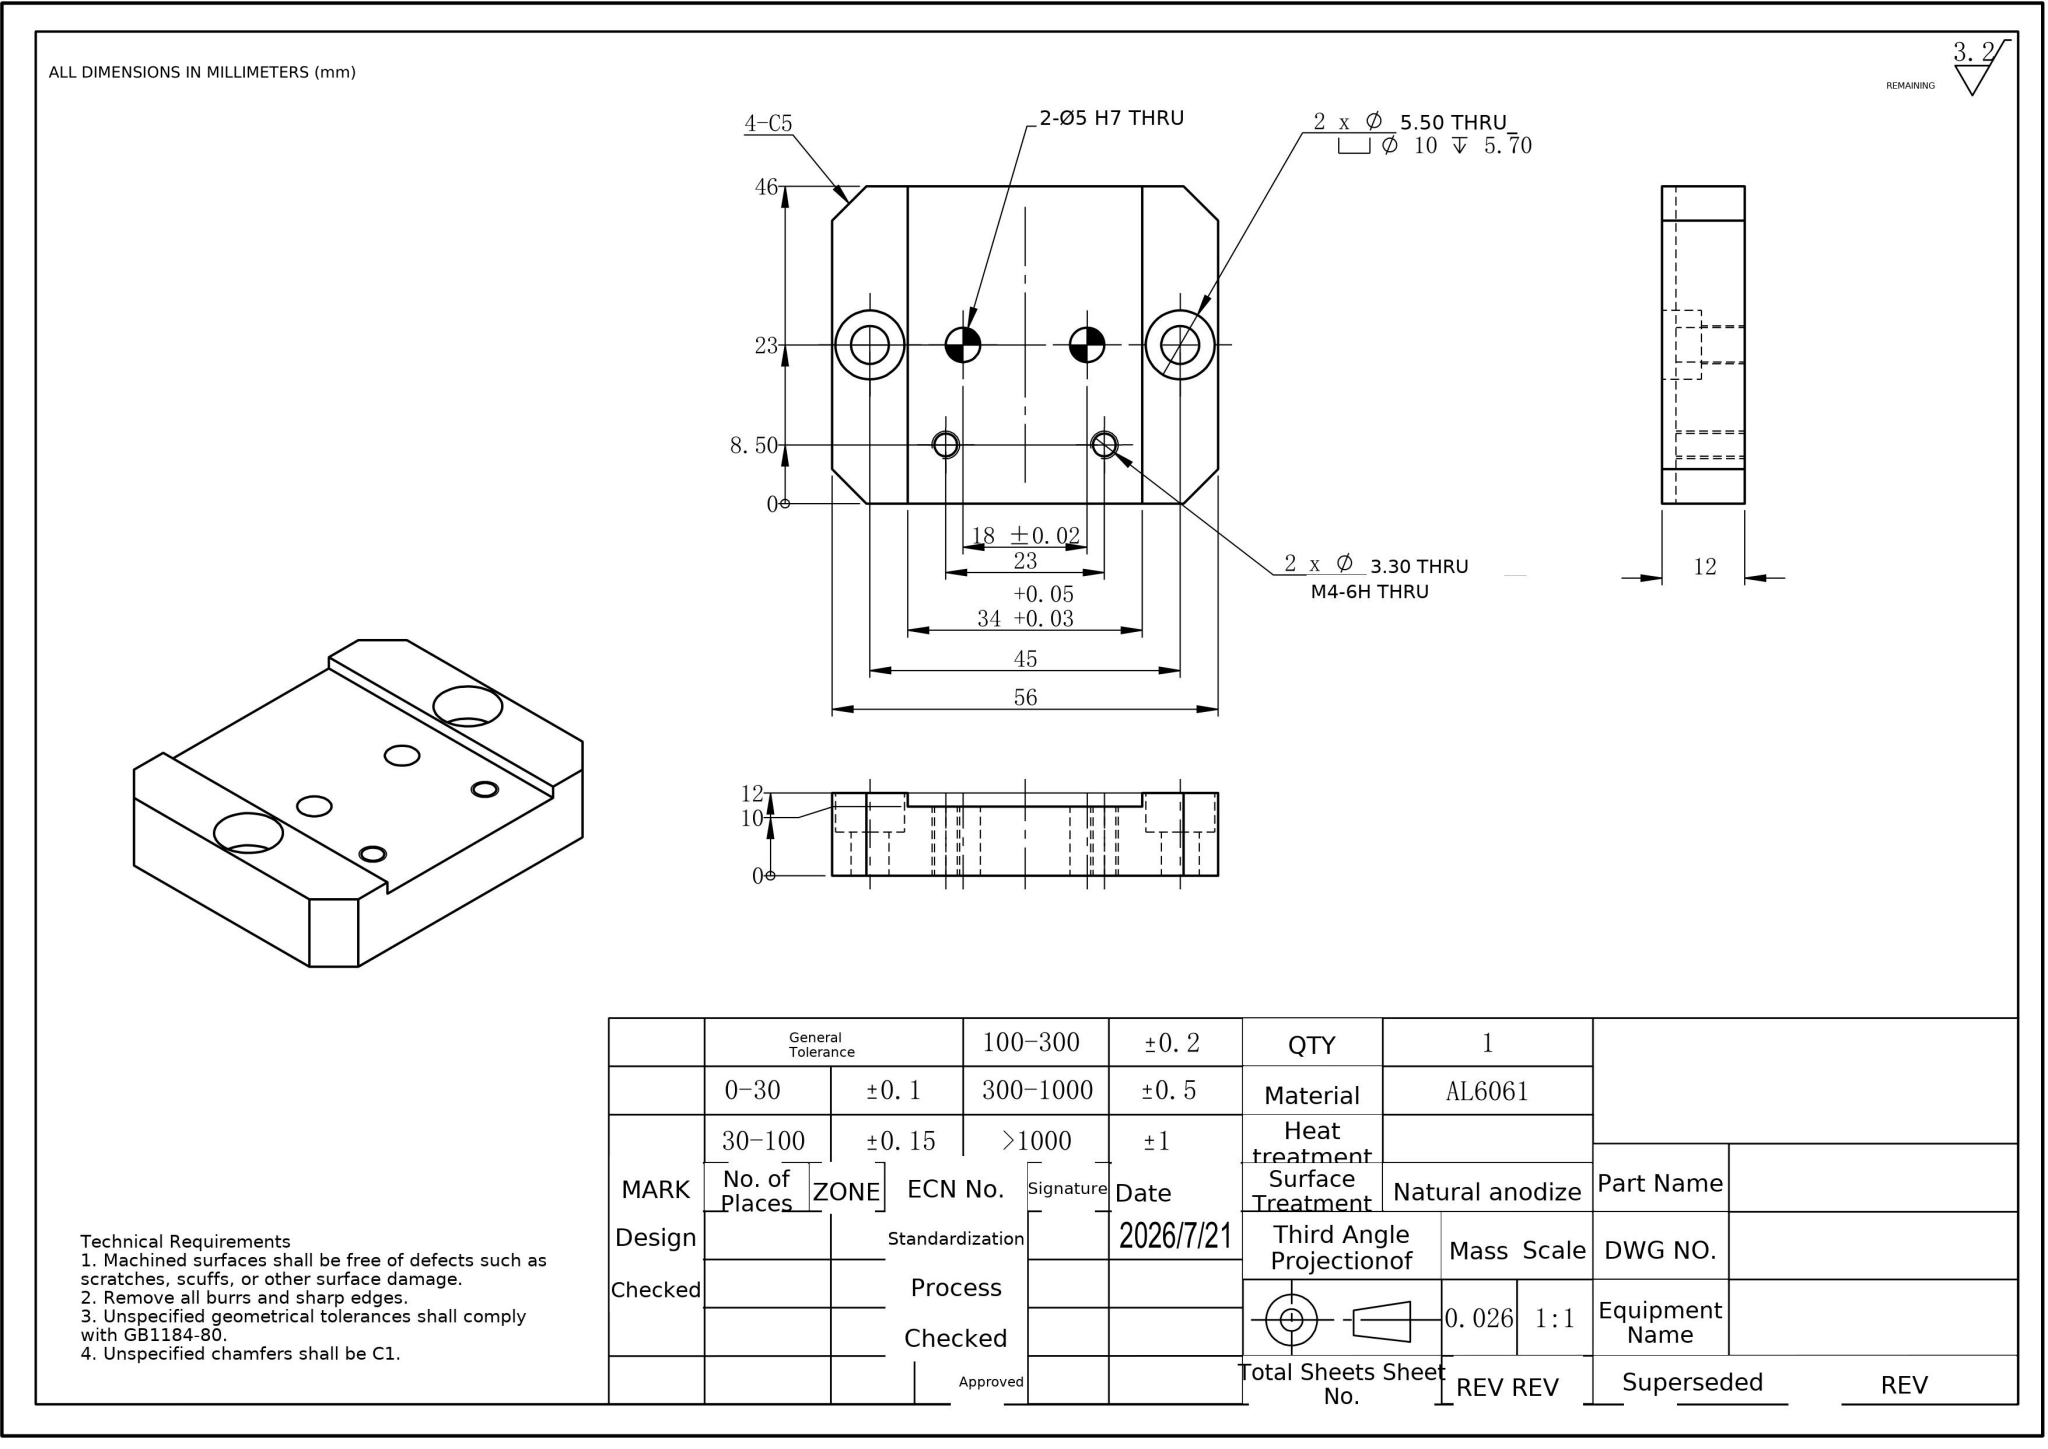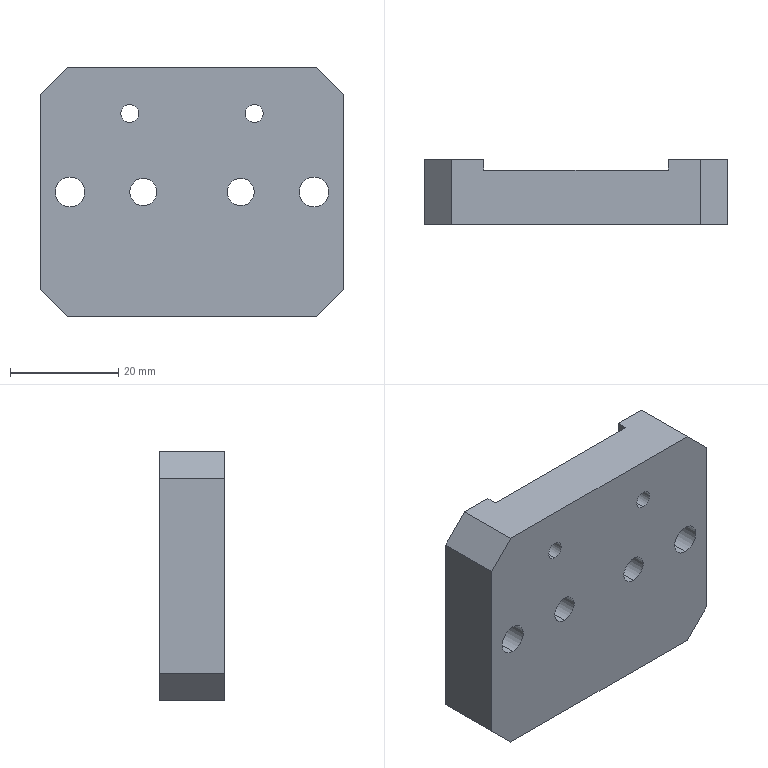Part | NX | mm | 1 solid | 32 faces | box 56 x 12 x 46 mm | volume 25426 mm3 | cylinder 16 | plane 16 | commonest cylinder face diameters 3.3 x4 5 x4 10 x4 5.5 x4
STEP:
#1=COLOUR_RGB('',0.7922,0.8196,0.9333);
#2=FILL_AREA_STYLE_COLOUR('',#1);
#3=FILL_AREA_STYLE('',(#2));
#4=SURFACE_STYLE_FILL_AREA(#3);
#5=SURFACE_SIDE_STYLE('',(#4));
#6=SURFACE_STYLE_USAGE(.BOTH.,#5);
#7=PRESENTATION_STYLE_ASSIGNMENT((#6));
#8=CARTESIAN_POINT('',(11.5,-5.,12.85));
#9=VERTEX_POINT('',#8);
#10=CARTESIAN_POINT('',(11.5,-5.,16.15));
#11=VERTEX_POINT('',#10);
#12=CARTESIAN_POINT('',(11.5,-5.,14.5));
#13=DIRECTION('',(0.,1.,0.));
#14=DIRECTION('',(0.,0.,1.));
#15=AXIS2_PLACEMENT_3D('',#12,#13,#14);
#16=CIRCLE('',#15,1.65);
#17=EDGE_CURVE('',#9,#11,#16,.T.);
#18=ORIENTED_EDGE('',*,*,#17,.F.);
#19=CARTESIAN_POINT('',(11.5,5.,12.85));
#20=VERTEX_POINT('',#19);
#21=CARTESIAN_POINT('',(11.5,7.,12.85));
#22=DIRECTION('',(0.,1.,0.));
#23=VECTOR('',#22,1000.);
#24=LINE('',#21,#23);
#25=EDGE_CURVE('',#9,#20,#24,.T.);
#26=ORIENTED_EDGE('',*,*,#25,.T.);
#27=CARTESIAN_POINT('',(11.5,5.,16.15));
#28=VERTEX_POINT('',#27);
#29=CARTESIAN_POINT('',(11.5,5.,14.5));
#30=DIRECTION('',(0.,-1.,0.));
#31=DIRECTION('',(0.,0.,-1.));
#32=AXIS2_PLACEMENT_3D('',#29,#30,#31);
#33=CIRCLE('',#32,1.65);
#34=EDGE_CURVE('',#28,#20,#33,.T.);
#35=ORIENTED_EDGE('',*,*,#34,.F.);
#36=CARTESIAN_POINT('',(11.5,7.,16.15));
#37=DIRECTION('',(0.,1.,0.));
#38=VECTOR('',#37,1000.);
#39=LINE('',#36,#38);
#40=EDGE_CURVE('',#11,#28,#39,.T.);
#41=ORIENTED_EDGE('',*,*,#40,.F.);
#42=EDGE_LOOP('',(#18,#26,#35,#41));
#43=FACE_OUTER_BOUND('',#42,.T.);
#44=CARTESIAN_POINT('',(11.5,7.,14.5));
#45=DIRECTION('',(0.,1.,0.));
#46=DIRECTION('',(0.,0.,1.));
#47=AXIS2_PLACEMENT_3D('',#44,#45,#46);
#48=CYLINDRICAL_SURFACE('',#47,1.65);
#49=ADVANCED_FACE('',(#43),#48,.F.);
#50=CARTESIAN_POINT('',(-11.5,-5.,12.85));
#51=VERTEX_POINT('',#50);
#52=CARTESIAN_POINT('',(-11.5,-5.,16.15));
#53=VERTEX_POINT('',#52);
#54=CARTESIAN_POINT('',(-11.5,-5.,14.5));
#55=DIRECTION('',(0.,1.,0.));
#56=DIRECTION('',(0.,0.,1.));
#57=AXIS2_PLACEMENT_3D('',#54,#55,#56);
#58=CIRCLE('',#57,1.65);
#59=EDGE_CURVE('',#51,#53,#58,.T.);
#60=ORIENTED_EDGE('',*,*,#59,.F.);
#61=CARTESIAN_POINT('',(-11.5,5.,12.85));
#62=VERTEX_POINT('',#61);
#63=CARTESIAN_POINT('',(-11.5,7.,12.85));
#64=DIRECTION('',(0.,1.,0.));
#65=VECTOR('',#64,1000.);
#66=LINE('',#63,#65);
#67=EDGE_CURVE('',#51,#62,#66,.T.);
#68=ORIENTED_EDGE('',*,*,#67,.T.);
#69=CARTESIAN_POINT('',(-11.5,5.,16.15));
#70=VERTEX_POINT('',#69);
#71=CARTESIAN_POINT('',(-11.5,5.,14.5));
#72=DIRECTION('',(0.,-1.,0.));
#73=DIRECTION('',(0.,0.,-1.));
#74=AXIS2_PLACEMENT_3D('',#71,#72,#73);
#75=CIRCLE('',#74,1.65);
#76=EDGE_CURVE('',#70,#62,#75,.T.);
#77=ORIENTED_EDGE('',*,*,#76,.F.);
#78=CARTESIAN_POINT('',(-11.5,7.,16.15));
#79=DIRECTION('',(0.,1.,0.));
#80=VECTOR('',#79,1000.);
#81=LINE('',#78,#80);
#82=EDGE_CURVE('',#53,#70,#81,.T.);
#83=ORIENTED_EDGE('',*,*,#82,.F.);
#84=EDGE_LOOP('',(#60,#68,#77,#83));
#85=FACE_OUTER_BOUND('',#84,.T.);
#86=CARTESIAN_POINT('',(-11.5,7.,14.5));
#87=DIRECTION('',(0.,1.,0.));
#88=DIRECTION('',(0.,0.,1.));
#89=AXIS2_PLACEMENT_3D('',#86,#87,#88);
#90=CYLINDRICAL_SURFACE('',#89,1.65);
#91=ADVANCED_FACE('',(#85),#90,.F.);
#92=CARTESIAN_POINT('',(-9.,-5.,2.5));
#93=VERTEX_POINT('',#92);
#94=CARTESIAN_POINT('',(-9.,-5.,-2.5));
#95=VERTEX_POINT('',#94);
#96=CARTESIAN_POINT('',(-9.,-5.,0.));
#97=DIRECTION('',(0.,-1.,0.));
#98=DIRECTION('',(0.,0.,-1.));
#99=AXIS2_PLACEMENT_3D('',#96,#97,#98);
#100=CIRCLE('',#99,2.5);
#101=EDGE_CURVE('',#93,#95,#100,.T.);
#102=ORIENTED_EDGE('',*,*,#101,.T.);
#103=CARTESIAN_POINT('',(-9.,5.,-2.5));
#104=VERTEX_POINT('',#103);
#105=CARTESIAN_POINT('',(-9.,-11.,-2.5));
#106=DIRECTION('',(0.,1.,0.));
#107=VECTOR('',#106,1000.);
#108=LINE('',#105,#107);
#109=EDGE_CURVE('',#95,#104,#108,.T.);
#110=ORIENTED_EDGE('',*,*,#109,.T.);
#111=CARTESIAN_POINT('',(-9.,5.,2.5));
#112=VERTEX_POINT('',#111);
#113=CARTESIAN_POINT('',(-9.,5.,0.));
#114=DIRECTION('',(0.,1.,0.));
#115=DIRECTION('',(0.,0.,-1.));
#116=AXIS2_PLACEMENT_3D('',#113,#114,#115);
#117=CIRCLE('',#116,2.5);
#118=EDGE_CURVE('',#104,#112,#117,.T.);
#119=ORIENTED_EDGE('',*,*,#118,.T.);
#120=CARTESIAN_POINT('',(-9.,-11.,2.5));
#121=DIRECTION('',(0.,1.,0.));
#122=VECTOR('',#121,1000.);
#123=LINE('',#120,#122);
#124=EDGE_CURVE('',#93,#112,#123,.T.);
#125=ORIENTED_EDGE('',*,*,#124,.F.);
#126=EDGE_LOOP('',(#102,#110,#119,#125));
#127=FACE_OUTER_BOUND('',#126,.T.);
#128=CARTESIAN_POINT('',(-9.,-11.,0.));
#129=DIRECTION('',(0.,1.,0.));
#130=DIRECTION('',(0.,0.,1.));
#131=AXIS2_PLACEMENT_3D('',#128,#129,#130);
#132=CYLINDRICAL_SURFACE('',#131,2.5);
#133=ADVANCED_FACE('',(#127),#132,.F.);
#134=CARTESIAN_POINT('',(9.,-5.,2.5));
#135=VERTEX_POINT('',#134);
#136=CARTESIAN_POINT('',(9.,-5.,-2.5));
#137=VERTEX_POINT('',#136);
#138=CARTESIAN_POINT('',(9.,-5.,0.));
#139=DIRECTION('',(0.,-1.,0.));
#140=DIRECTION('',(0.,0.,-1.));
#141=AXIS2_PLACEMENT_3D('',#138,#139,#140);
#142=CIRCLE('',#141,2.5);
#143=EDGE_CURVE('',#135,#137,#142,.T.);
#144=ORIENTED_EDGE('',*,*,#143,.T.);
#145=CARTESIAN_POINT('',(9.,5.,-2.5));
#146=VERTEX_POINT('',#145);
#147=CARTESIAN_POINT('',(9.,-11.,-2.5));
#148=DIRECTION('',(0.,1.,0.));
#149=VECTOR('',#148,1000.);
#150=LINE('',#147,#149);
#151=EDGE_CURVE('',#137,#146,#150,.T.);
#152=ORIENTED_EDGE('',*,*,#151,.T.);
#153=CARTESIAN_POINT('',(9.,5.,2.5));
#154=VERTEX_POINT('',#153);
#155=CARTESIAN_POINT('',(9.,5.,0.));
#156=DIRECTION('',(0.,1.,0.));
#157=DIRECTION('',(0.,0.,1.));
#158=AXIS2_PLACEMENT_3D('',#155,#156,#157);
#159=CIRCLE('',#158,2.5);
#160=EDGE_CURVE('',#146,#154,#159,.T.);
#161=ORIENTED_EDGE('',*,*,#160,.T.);
#162=CARTESIAN_POINT('',(9.,-11.,2.5));
#163=DIRECTION('',(0.,1.,0.));
#164=VECTOR('',#163,1000.);
#165=LINE('',#162,#164);
#166=EDGE_CURVE('',#135,#154,#165,.T.);
#167=ORIENTED_EDGE('',*,*,#166,.F.);
#168=EDGE_LOOP('',(#144,#152,#161,#167));
#169=FACE_OUTER_BOUND('',#168,.T.);
#170=CARTESIAN_POINT('',(9.,-11.,0.));
#171=DIRECTION('',(0.,1.,0.));
#172=DIRECTION('',(0.,0.,1.));
#173=AXIS2_PLACEMENT_3D('',#170,#171,#172);
#174=CYLINDRICAL_SURFACE('',#173,2.5);
#175=ADVANCED_FACE('',(#169),#174,.F.);
#176=CARTESIAN_POINT('',(22.5,1.3,-5.));
#177=VERTEX_POINT('',#176);
#178=CARTESIAN_POINT('',(22.5,1.3,5.));
#179=VERTEX_POINT('',#178);
#180=CARTESIAN_POINT('',(22.5,1.3,-0.));
#181=DIRECTION('',(0.,1.,0.));
#182=DIRECTION('',(0.,0.,1.));
#183=AXIS2_PLACEMENT_3D('',#180,#181,#182);
#184=CIRCLE('',#183,5.);
#185=EDGE_CURVE('',#177,#179,#184,.T.);
#186=ORIENTED_EDGE('',*,*,#185,.F.);
#187=CARTESIAN_POINT('',(22.5,7.,-5.));
#188=VERTEX_POINT('',#187);
#189=CARTESIAN_POINT('',(22.5,7.,-5.));
#190=DIRECTION('',(0.,1.,0.));
#191=VECTOR('',#190,1000.);
#192=LINE('',#189,#191);
#193=EDGE_CURVE('',#177,#188,#192,.T.);
#194=ORIENTED_EDGE('',*,*,#193,.T.);
#195=CARTESIAN_POINT('',(22.5,7.,5.));
#196=VERTEX_POINT('',#195);
#197=CARTESIAN_POINT('',(22.5,7.,-0.));
#198=DIRECTION('',(0.,1.,0.));
#199=DIRECTION('',(0.,0.,1.));
#200=AXIS2_PLACEMENT_3D('',#197,#198,#199);
#201=CIRCLE('',#200,5.);
#202=EDGE_CURVE('',#188,#196,#201,.T.);
#203=ORIENTED_EDGE('',*,*,#202,.T.);
#204=CARTESIAN_POINT('',(22.5,7.,5.));
#205=DIRECTION('',(0.,1.,0.));
#206=VECTOR('',#205,1000.);
#207=LINE('',#204,#206);
#208=EDGE_CURVE('',#179,#196,#207,.T.);
#209=ORIENTED_EDGE('',*,*,#208,.F.);
#210=EDGE_LOOP('',(#186,#194,#203,#209));
#211=FACE_OUTER_BOUND('',#210,.T.);
#212=CARTESIAN_POINT('',(22.5,7.,-0.));
#213=DIRECTION('',(0.,1.,0.));
#214=DIRECTION('',(0.,0.,1.));
#215=AXIS2_PLACEMENT_3D('',#212,#213,#214);
#216=CYLINDRICAL_SURFACE('',#215,5.);
#217=ADVANCED_FACE('',(#211),#216,.F.);
#218=CARTESIAN_POINT('',(22.5,-5.,-2.75));
#219=VERTEX_POINT('',#218);
#220=CARTESIAN_POINT('',(22.5,-5.,2.75));
#221=VERTEX_POINT('',#220);
#222=CARTESIAN_POINT('',(22.5,-5.,-0.));
#223=DIRECTION('',(0.,1.,0.));
#224=DIRECTION('',(0.,0.,1.));
#225=AXIS2_PLACEMENT_3D('',#222,#223,#224);
#226=CIRCLE('',#225,2.75);
#227=EDGE_CURVE('',#219,#221,#226,.T.);
#228=ORIENTED_EDGE('',*,*,#227,.F.);
#229=CARTESIAN_POINT('',(22.5,1.3,-2.75));
#230=VERTEX_POINT('',#229);
#231=CARTESIAN_POINT('',(22.5,7.,-2.75));
#232=DIRECTION('',(0.,1.,0.));
#233=VECTOR('',#232,1000.);
#234=LINE('',#231,#233);
#235=EDGE_CURVE('',#219,#230,#234,.T.);
#236=ORIENTED_EDGE('',*,*,#235,.T.);
#237=CARTESIAN_POINT('',(22.5,1.3,2.75));
#238=VERTEX_POINT('',#237);
#239=CARTESIAN_POINT('',(22.5,1.3,-0.));
#240=DIRECTION('',(0.,1.,0.));
#241=DIRECTION('',(0.,0.,1.));
#242=AXIS2_PLACEMENT_3D('',#239,#240,#241);
#243=CIRCLE('',#242,2.75);
#244=EDGE_CURVE('',#230,#238,#243,.T.);
#245=ORIENTED_EDGE('',*,*,#244,.T.);
#246=CARTESIAN_POINT('',(22.5,7.,2.75));
#247=DIRECTION('',(0.,1.,0.));
#248=VECTOR('',#247,1000.);
#249=LINE('',#246,#248);
#250=EDGE_CURVE('',#221,#238,#249,.T.);
#251=ORIENTED_EDGE('',*,*,#250,.F.);
#252=EDGE_LOOP('',(#228,#236,#245,#251));
#253=FACE_OUTER_BOUND('',#252,.T.);
#254=CARTESIAN_POINT('',(22.5,7.,-0.));
#255=DIRECTION('',(0.,1.,0.));
#256=DIRECTION('',(0.,0.,1.));
#257=AXIS2_PLACEMENT_3D('',#254,#255,#256);
#258=CYLINDRICAL_SURFACE('',#257,2.75);
#259=ADVANCED_FACE('',(#253),#258,.F.);
#260=CARTESIAN_POINT('',(-22.5,1.3,-5.));
#261=VERTEX_POINT('',#260);
#262=CARTESIAN_POINT('',(-22.5,1.3,5.));
#263=VERTEX_POINT('',#262);
#264=CARTESIAN_POINT('',(-22.5,1.3,0.));
#265=DIRECTION('',(0.,1.,0.));
#266=DIRECTION('',(0.,0.,1.));
#267=AXIS2_PLACEMENT_3D('',#264,#265,#266);
#268=CIRCLE('',#267,5.);
#269=EDGE_CURVE('',#261,#263,#268,.T.);
#270=ORIENTED_EDGE('',*,*,#269,.F.);
#271=CARTESIAN_POINT('',(-22.5,7.,-5.));
#272=VERTEX_POINT('',#271);
#273=CARTESIAN_POINT('',(-22.5,7.,-5.));
#274=DIRECTION('',(0.,1.,0.));
#275=VECTOR('',#274,1000.);
#276=LINE('',#273,#275);
#277=EDGE_CURVE('',#261,#272,#276,.T.);
#278=ORIENTED_EDGE('',*,*,#277,.T.);
#279=CARTESIAN_POINT('',(-22.5,7.,5.));
#280=VERTEX_POINT('',#279);
#281=CARTESIAN_POINT('',(-22.5,7.,0.));
#282=DIRECTION('',(0.,1.,0.));
#283=DIRECTION('',(0.,0.,1.));
#284=AXIS2_PLACEMENT_3D('',#281,#282,#283);
#285=CIRCLE('',#284,5.);
#286=EDGE_CURVE('',#272,#280,#285,.T.);
#287=ORIENTED_EDGE('',*,*,#286,.T.);
#288=CARTESIAN_POINT('',(-22.5,7.,5.));
#289=DIRECTION('',(0.,1.,0.));
#290=VECTOR('',#289,1000.);
#291=LINE('',#288,#290);
#292=EDGE_CURVE('',#263,#280,#291,.T.);
#293=ORIENTED_EDGE('',*,*,#292,.F.);
#294=EDGE_LOOP('',(#270,#278,#287,#293));
#295=FACE_OUTER_BOUND('',#294,.T.);
#296=CARTESIAN_POINT('',(-22.5,7.,0.));
#297=DIRECTION('',(0.,1.,0.));
#298=DIRECTION('',(0.,0.,1.));
#299=AXIS2_PLACEMENT_3D('',#296,#297,#298);
#300=CYLINDRICAL_SURFACE('',#299,5.);
#301=ADVANCED_FACE('',(#295),#300,.F.);
#302=CARTESIAN_POINT('',(-22.5,-5.,-2.75));
#303=VERTEX_POINT('',#302);
#304=CARTESIAN_POINT('',(-22.5,-5.,2.75));
#305=VERTEX_POINT('',#304);
#306=CARTESIAN_POINT('',(-22.5,-5.,0.));
#307=DIRECTION('',(0.,1.,0.));
#308=DIRECTION('',(0.,0.,1.));
#309=AXIS2_PLACEMENT_3D('',#306,#307,#308);
#310=CIRCLE('',#309,2.75);
#311=EDGE_CURVE('',#303,#305,#310,.T.);
#312=ORIENTED_EDGE('',*,*,#311,.F.);
#313=CARTESIAN_POINT('',(-22.5,1.3,-2.75));
#314=VERTEX_POINT('',#313);
#315=CARTESIAN_POINT('',(-22.5,7.,-2.75));
#316=DIRECTION('',(0.,1.,0.));
#317=VECTOR('',#316,1000.);
#318=LINE('',#315,#317);
#319=EDGE_CURVE('',#303,#314,#318,.T.);
#320=ORIENTED_EDGE('',*,*,#319,.T.);
#321=CARTESIAN_POINT('',(-22.5,1.3,2.75));
#322=VERTEX_POINT('',#321);
#323=CARTESIAN_POINT('',(-22.5,1.3,0.));
#324=DIRECTION('',(0.,1.,0.));
#325=DIRECTION('',(0.,0.,1.));
#326=AXIS2_PLACEMENT_3D('',#323,#324,#325);
#327=CIRCLE('',#326,2.75);
#328=EDGE_CURVE('',#314,#322,#327,.T.);
#329=ORIENTED_EDGE('',*,*,#328,.T.);
#330=CARTESIAN_POINT('',(-22.5,7.,2.75));
#331=DIRECTION('',(0.,1.,0.));
#332=VECTOR('',#331,1000.);
#333=LINE('',#330,#332);
#334=EDGE_CURVE('',#305,#322,#333,.T.);
#335=ORIENTED_EDGE('',*,*,#334,.F.);
#336=EDGE_LOOP('',(#312,#320,#329,#335));
#337=FACE_OUTER_BOUND('',#336,.T.);
#338=CARTESIAN_POINT('',(-22.5,7.,0.));
#339=DIRECTION('',(0.,1.,0.));
#340=DIRECTION('',(0.,0.,1.));
#341=AXIS2_PLACEMENT_3D('',#338,#339,#340);
#342=CYLINDRICAL_SURFACE('',#341,2.75);
#343=ADVANCED_FACE('',(#337),#342,.F.);
#344=ORIENTED_EDGE('',*,*,#34,.T.);
#345=CARTESIAN_POINT('',(11.5,5.,14.5));
#346=DIRECTION('',(0.,-1.,0.));
#347=DIRECTION('',(0.,0.,-1.));
#348=AXIS2_PLACEMENT_3D('',#345,#346,#347);
#349=CIRCLE('',#348,1.65);
#350=EDGE_CURVE('',#20,#28,#349,.T.);
#351=ORIENTED_EDGE('',*,*,#350,.T.);
#352=EDGE_LOOP('',(#344,#351));
#353=FACE_BOUND('',#352,.T.);
#354=ORIENTED_EDGE('',*,*,#76,.T.);
#355=CARTESIAN_POINT('',(-11.5,5.,14.5));
#356=DIRECTION('',(0.,-1.,0.));
#357=DIRECTION('',(0.,0.,-1.));
#358=AXIS2_PLACEMENT_3D('',#355,#356,#357);
#359=CIRCLE('',#358,1.65);
#360=EDGE_CURVE('',#62,#70,#359,.T.);
#361=ORIENTED_EDGE('',*,*,#360,.T.);
#362=EDGE_LOOP('',(#354,#361));
#363=FACE_BOUND('',#362,.T.);
#364=CARTESIAN_POINT('',(-9.,5.,0.));
#365=DIRECTION('',(0.,1.,0.));
#366=DIRECTION('',(0.,0.,-1.));
#367=AXIS2_PLACEMENT_3D('',#364,#365,#366);
#368=CIRCLE('',#367,2.5);
#369=EDGE_CURVE('',#112,#104,#368,.T.);
#370=ORIENTED_EDGE('',*,*,#369,.F.);
#371=ORIENTED_EDGE('',*,*,#118,.F.);
#372=EDGE_LOOP('',(#370,#371));
#373=FACE_BOUND('',#372,.T.);
#374=CARTESIAN_POINT('',(9.,5.,0.));
#375=DIRECTION('',(0.,1.,0.));
#376=DIRECTION('',(0.,0.,1.));
#377=AXIS2_PLACEMENT_3D('',#374,#375,#376);
#378=CIRCLE('',#377,2.5);
#379=EDGE_CURVE('',#154,#146,#378,.T.);
#380=ORIENTED_EDGE('',*,*,#379,.F.);
#381=ORIENTED_EDGE('',*,*,#160,.F.);
#382=EDGE_LOOP('',(#380,#381));
#383=FACE_BOUND('',#382,.T.);
#384=CARTESIAN_POINT('',(17.,5.,-23.));
#385=VERTEX_POINT('',#384);
#386=CARTESIAN_POINT('',(-17.,5.,-23.));
#387=VERTEX_POINT('',#386);
#388=CARTESIAN_POINT('',(-28.,5.,-23.));
#389=DIRECTION('',(-1.,0.,0.));
#390=VECTOR('',#389,1000.);
#391=LINE('',#388,#390);
#392=EDGE_CURVE('',#385,#387,#391,.T.);
#393=ORIENTED_EDGE('',*,*,#392,.T.);
#394=CARTESIAN_POINT('',(-17.,5.,23.));
#395=VERTEX_POINT('',#394);
#396=CARTESIAN_POINT('',(-17.,5.,-23.));
#397=DIRECTION('',(-0.,0.,1.));
#398=VECTOR('',#397,1000.);
#399=LINE('',#396,#398);
#400=EDGE_CURVE('',#387,#395,#399,.T.);
#401=ORIENTED_EDGE('',*,*,#400,.T.);
#402=CARTESIAN_POINT('',(17.,5.,23.));
#403=VERTEX_POINT('',#402);
#404=CARTESIAN_POINT('',(-28.,5.,23.));
#405=DIRECTION('',(1.,0.,0.));
#406=VECTOR('',#405,1000.);
#407=LINE('',#404,#406);
#408=EDGE_CURVE('',#395,#403,#407,.T.);
#409=ORIENTED_EDGE('',*,*,#408,.T.);
#410=CARTESIAN_POINT('',(17.,5.,-23.));
#411=DIRECTION('',(0.,0.,1.));
#412=VECTOR('',#411,1000.);
#413=LINE('',#410,#412);
#414=EDGE_CURVE('',#385,#403,#413,.T.);
#415=ORIENTED_EDGE('',*,*,#414,.F.);
#416=EDGE_LOOP('',(#393,#401,#409,#415));
#417=FACE_OUTER_BOUND('',#416,.T.);
#418=CARTESIAN_POINT('',(0.,5.,0.));
#419=DIRECTION('',(0.,-1.,0.));
#420=DIRECTION('',(0.,0.,-1.));
#421=AXIS2_PLACEMENT_3D('',#418,#419,#420);
#422=PLANE('',#421);
#423=ADVANCED_FACE('',(#353,#363,#373,#383,#417),#422,.F.);
#424=CARTESIAN_POINT('',(28.,7.,18.));
#425=VERTEX_POINT('',#424);
#426=CARTESIAN_POINT('',(28.,7.,-18.));
#427=VERTEX_POINT('',#426);
#428=CARTESIAN_POINT('',(28.,7.,-23.));
#429=DIRECTION('',(-0.,0.,-1.));
#430=VECTOR('',#429,1000.);
#431=LINE('',#428,#430);
#432=EDGE_CURVE('',#425,#427,#431,.T.);
#433=ORIENTED_EDGE('',*,*,#432,.F.);
#434=CARTESIAN_POINT('',(28.,-5.,18.));
#435=VERTEX_POINT('',#434);
#436=CARTESIAN_POINT('',(28.,5.,18.));
#437=DIRECTION('',(0.,-1.,0.));
#438=VECTOR('',#437,1000.);
#439=LINE('',#436,#438);
#440=EDGE_CURVE('',#425,#435,#439,.T.);
#441=ORIENTED_EDGE('',*,*,#440,.T.);
#442=CARTESIAN_POINT('',(28.,-5.,-18.));
#443=VERTEX_POINT('',#442);
#444=CARTESIAN_POINT('',(28.,-5.,23.));
#445=DIRECTION('',(0.,0.,-1.));
#446=VECTOR('',#445,1000.);
#447=LINE('',#444,#446);
#448=EDGE_CURVE('',#435,#443,#447,.T.);
#449=ORIENTED_EDGE('',*,*,#448,.T.);
#450=CARTESIAN_POINT('',(28.,5.,-18.));
#451=DIRECTION('',(0.,1.,0.));
#452=VECTOR('',#451,1000.);
#453=LINE('',#450,#452);
#454=EDGE_CURVE('',#443,#427,#453,.T.);
#455=ORIENTED_EDGE('',*,*,#454,.T.);
#456=EDGE_LOOP('',(#433,#441,#449,#455));
#457=FACE_OUTER_BOUND('',#456,.T.);
#458=CARTESIAN_POINT('',(28.,5.,23.));
#459=DIRECTION('',(-1.,0.,0.));
#460=DIRECTION('',(0.,0.,1.));
#461=AXIS2_PLACEMENT_3D('',#458,#459,#460);
#462=PLANE('',#461);
#463=ADVANCED_FACE('',(#457),#462,.F.);
#464=CARTESIAN_POINT('',(23.,-5.,-23.));
#465=VERTEX_POINT('',#464);
#466=CARTESIAN_POINT('',(-23.,-5.,-23.));
#467=VERTEX_POINT('',#466);
#468=CARTESIAN_POINT('',(-28.,-5.,-23.));
#469=DIRECTION('',(-1.,0.,0.));
#470=VECTOR('',#469,1000.);
#471=LINE('',#468,#470);
#472=EDGE_CURVE('',#465,#467,#471,.T.);
#473=ORIENTED_EDGE('',*,*,#472,.T.);
#474=CARTESIAN_POINT('',(-23.,7.,-23.));
#475=VERTEX_POINT('',#474);
#476=CARTESIAN_POINT('',(-23.,5.,-23.));
#477=DIRECTION('',(0.,1.,0.));
#478=VECTOR('',#477,1000.);
#479=LINE('',#476,#478);
#480=EDGE_CURVE('',#467,#475,#479,.T.);
#481=ORIENTED_EDGE('',*,*,#480,.T.);
#482=CARTESIAN_POINT('',(-17.,7.,-23.));
#483=VERTEX_POINT('',#482);
#484=CARTESIAN_POINT('',(-28.,7.,-23.));
#485=DIRECTION('',(1.,0.,0.));
#486=VECTOR('',#485,1000.);
#487=LINE('',#484,#486);
#488=EDGE_CURVE('',#475,#483,#487,.T.);
#489=ORIENTED_EDGE('',*,*,#488,.T.);
#490=CARTESIAN_POINT('',(-17.,7.,-23.));
#491=DIRECTION('',(0.,-1.,0.));
#492=VECTOR('',#491,1000.);
#493=LINE('',#490,#492);
#494=EDGE_CURVE('',#483,#387,#493,.T.);
#495=ORIENTED_EDGE('',*,*,#494,.T.);
#496=ORIENTED_EDGE('',*,*,#392,.F.);
#497=CARTESIAN_POINT('',(17.,7.,-23.));
#498=VERTEX_POINT('',#497);
#499=CARTESIAN_POINT('',(17.,7.,-23.));
#500=DIRECTION('',(0.,-1.,0.));
#501=VECTOR('',#500,1000.);
#502=LINE('',#499,#501);
#503=EDGE_CURVE('',#498,#385,#502,.T.);
#504=ORIENTED_EDGE('',*,*,#503,.F.);
#505=CARTESIAN_POINT('',(23.,7.,-23.));
#506=VERTEX_POINT('',#505);
#507=CARTESIAN_POINT('',(28.,7.,-23.));
#508=DIRECTION('',(-1.,0.,0.));
#509=VECTOR('',#508,1000.);
#510=LINE('',#507,#509);
#511=EDGE_CURVE('',#506,#498,#510,.T.);
#512=ORIENTED_EDGE('',*,*,#511,.F.);
#513=CARTESIAN_POINT('',(23.,5.,-23.));
#514=DIRECTION('',(0.,-1.,0.));
#515=VECTOR('',#514,1000.);
#516=LINE('',#513,#515);
#517=EDGE_CURVE('',#506,#465,#516,.T.);
#518=ORIENTED_EDGE('',*,*,#517,.T.);
#519=EDGE_LOOP('',(#473,#481,#489,#495,#496,#504,#512,#518));
#520=FACE_OUTER_BOUND('',#519,.T.);
#521=CARTESIAN_POINT('',(-28.,5.,-23.));
#522=DIRECTION('',(0.,0.,1.));
#523=DIRECTION('',(1.,0.,0.));
#524=AXIS2_PLACEMENT_3D('',#521,#522,#523);
#525=PLANE('',#524);
#526=ADVANCED_FACE('',(#520),#525,.F.);
#527=CARTESIAN_POINT('',(-28.,-5.,-18.));
#528=VERTEX_POINT('',#527);
#529=CARTESIAN_POINT('',(-28.,-5.,18.));
#530=VERTEX_POINT('',#529);
#531=CARTESIAN_POINT('',(-28.,-5.,23.));
#532=DIRECTION('',(0.,0.,1.));
#533=VECTOR('',#532,1000.);
#534=LINE('',#531,#533);
#535=EDGE_CURVE('',#528,#530,#534,.T.);
#536=ORIENTED_EDGE('',*,*,#535,.T.);
#537=CARTESIAN_POINT('',(-28.,7.,18.));
#538=VERTEX_POINT('',#537);
#539=CARTESIAN_POINT('',(-28.,5.,18.));
#540=DIRECTION('',(0.,1.,0.));
#541=VECTOR('',#540,1000.);
#542=LINE('',#539,#541);
#543=EDGE_CURVE('',#530,#538,#542,.T.);
#544=ORIENTED_EDGE('',*,*,#543,.T.);
#545=CARTESIAN_POINT('',(-28.,7.,-18.));
#546=VERTEX_POINT('',#545);
#547=CARTESIAN_POINT('',(-28.,7.,-23.));
#548=DIRECTION('',(0.,0.,-1.));
#549=VECTOR('',#548,1000.);
#550=LINE('',#547,#549);
#551=EDGE_CURVE('',#538,#546,#550,.T.);
#552=ORIENTED_EDGE('',*,*,#551,.T.);
#553=CARTESIAN_POINT('',(-28.,5.,-18.));
#554=DIRECTION('',(0.,-1.,0.));
#555=VECTOR('',#554,1000.);
#556=LINE('',#553,#555);
#557=EDGE_CURVE('',#546,#528,#556,.T.);
#558=ORIENTED_EDGE('',*,*,#557,.T.);
#559=EDGE_LOOP('',(#536,#544,#552,#558));
#560=FACE_OUTER_BOUND('',#559,.T.);
#561=CARTESIAN_POINT('',(-28.,5.,23.));
#562=DIRECTION('',(1.,0.,0.));
#563=DIRECTION('',(0.,0.,-1.));
#564=AXIS2_PLACEMENT_3D('',#561,#562,#563);
#565=PLANE('',#564);
#566=ADVANCED_FACE('',(#560),#565,.F.);
#567=CARTESIAN_POINT('',(-17.,7.,23.));
#568=VERTEX_POINT('',#567);
#569=CARTESIAN_POINT('',(-23.,7.,23.));
#570=VERTEX_POINT('',#569);
#571=CARTESIAN_POINT('',(-28.,7.,23.));
#572=DIRECTION('',(-1.,0.,0.));
#573=VECTOR('',#572,1000.);
#574=LINE('',#571,#573);
#575=EDGE_CURVE('',#568,#570,#574,.T.);
#576=ORIENTED_EDGE('',*,*,#575,.T.);
#577=CARTESIAN_POINT('',(-23.,-5.,23.));
#578=VERTEX_POINT('',#577);
#579=CARTESIAN_POINT('',(-23.,5.,23.));
#580=DIRECTION('',(0.,-1.,0.));
#581=VECTOR('',#580,1000.);
#582=LINE('',#579,#581);
#583=EDGE_CURVE('',#570,#578,#582,.T.);
#584=ORIENTED_EDGE('',*,*,#583,.T.);
#585=CARTESIAN_POINT('',(23.,-5.,23.));
#586=VERTEX_POINT('',#585);
#587=CARTESIAN_POINT('',(-28.,-5.,23.));
#588=DIRECTION('',(1.,0.,0.));
#589=VECTOR('',#588,1000.);
#590=LINE('',#587,#589);
#591=EDGE_CURVE('',#578,#586,#590,.T.);
#592=ORIENTED_EDGE('',*,*,#591,.T.);
#593=CARTESIAN_POINT('',(23.,7.,23.));
#594=VERTEX_POINT('',#593);
#595=CARTESIAN_POINT('',(23.,5.,23.));
#596=DIRECTION('',(0.,1.,0.));
#597=VECTOR('',#596,1000.);
#598=LINE('',#595,#597);
#599=EDGE_CURVE('',#586,#594,#598,.T.);
#600=ORIENTED_EDGE('',*,*,#599,.T.);
#601=CARTESIAN_POINT('',(17.,7.,23.));
#602=VERTEX_POINT('',#601);
#603=CARTESIAN_POINT('',(28.,7.,23.));
#604=DIRECTION('',(1.,0.,0.));
#605=VECTOR('',#604,1000.);
#606=LINE('',#603,#605);
#607=EDGE_CURVE('',#602,#594,#606,.T.);
#608=ORIENTED_EDGE('',*,*,#607,.F.);
#609=CARTESIAN_POINT('',(17.,7.,23.));
#610=DIRECTION('',(0.,-1.,0.));
#611=VECTOR('',#610,1000.);
#612=LINE('',#609,#611);
#613=EDGE_CURVE('',#602,#403,#612,.T.);
#614=ORIENTED_EDGE('',*,*,#613,.T.);
#615=ORIENTED_EDGE('',*,*,#408,.F.);
#616=CARTESIAN_POINT('',(-17.,7.,23.));
#617=DIRECTION('',(0.,-1.,0.));
#618=VECTOR('',#617,1000.);
#619=LINE('',#616,#618);
#620=EDGE_CURVE('',#568,#395,#619,.T.);
#621=ORIENTED_EDGE('',*,*,#620,.F.);
#622=EDGE_LOOP('',(#576,#584,#592,#600,#608,#614,#615,#621));
#623=FACE_OUTER_BOUND('',#622,.T.);
#624=CARTESIAN_POINT('',(-28.,5.,23.));
#625=DIRECTION('',(0.,0.,-1.));
#626=DIRECTION('',(-1.,0.,0.));
#627=AXIS2_PLACEMENT_3D('',#624,#625,#626);
#628=PLANE('',#627);
#629=ADVANCED_FACE('',(#623),#628,.F.);
#630=CARTESIAN_POINT('',(11.5,-5.,14.5));
#631=DIRECTION('',(0.,1.,0.));
#632=DIRECTION('',(0.,0.,1.));
#633=AXIS2_PLACEMENT_3D('',#630,#631,#632);
#634=CIRCLE('',#633,1.65);
#635=EDGE_CURVE('',#11,#9,#634,.T.);
#636=ORIENTED_EDGE('',*,*,#635,.T.);
#637=ORIENTED_EDGE('',*,*,#17,.T.);
#638=EDGE_LOOP('',(#636,#637));
#639=FACE_BOUND('',#638,.T.);
#640=CARTESIAN_POINT('',(-11.5,-5.,14.5));
#641=DIRECTION('',(0.,1.,0.));
#642=DIRECTION('',(0.,0.,1.));
#643=AXIS2_PLACEMENT_3D('',#640,#641,#642);
#644=CIRCLE('',#643,1.65);
#645=EDGE_CURVE('',#53,#51,#644,.T.);
#646=ORIENTED_EDGE('',*,*,#645,.T.);
#647=ORIENTED_EDGE('',*,*,#59,.T.);
#648=EDGE_LOOP('',(#646,#647));
#649=FACE_BOUND('',#648,.T.);
#650=ORIENTED_EDGE('',*,*,#101,.F.);
#651=CARTESIAN_POINT('',(-9.,-5.,0.));
#652=DIRECTION('',(0.,-1.,0.));
#653=DIRECTION('',(0.,0.,-1.));
#654=AXIS2_PLACEMENT_3D('',#651,#652,#653);
#655=CIRCLE('',#654,2.5);
#656=EDGE_CURVE('',#95,#93,#655,.T.);
#657=ORIENTED_EDGE('',*,*,#656,.F.);
#658=EDGE_LOOP('',(#650,#657));
#659=FACE_BOUND('',#658,.T.);
#660=ORIENTED_EDGE('',*,*,#143,.F.);
#661=CARTESIAN_POINT('',(9.,-5.,0.));
#662=DIRECTION('',(0.,-1.,0.));
#663=DIRECTION('',(0.,0.,-1.));
#664=AXIS2_PLACEMENT_3D('',#661,#662,#663);
#665=CIRCLE('',#664,2.5);
#666=EDGE_CURVE('',#137,#135,#665,.T.);
#667=ORIENTED_EDGE('',*,*,#666,.F.);
#668=EDGE_LOOP('',(#660,#667));
#669=FACE_BOUND('',#668,.T.);
#670=CARTESIAN_POINT('',(22.5,-5.,-0.));
#671=DIRECTION('',(0.,1.,0.));
#672=DIRECTION('',(0.,0.,1.));
#673=AXIS2_PLACEMENT_3D('',#670,#671,#672);
#674=CIRCLE('',#673,2.75);
#675=EDGE_CURVE('',#221,#219,#674,.T.);
#676=ORIENTED_EDGE('',*,*,#675,.T.);
#677=ORIENTED_EDGE('',*,*,#227,.T.);
#678=EDGE_LOOP('',(#676,#677));
#679=FACE_BOUND('',#678,.T.);
#680=CARTESIAN_POINT('',(-22.5,-5.,0.));
#681=DIRECTION('',(0.,1.,0.));
#682=DIRECTION('',(0.,0.,1.));
#683=AXIS2_PLACEMENT_3D('',#680,#681,#682);
#684=CIRCLE('',#683,2.75);
#685=EDGE_CURVE('',#305,#303,#684,.T.);
#686=ORIENTED_EDGE('',*,*,#685,.T.);
#687=ORIENTED_EDGE('',*,*,#311,.T.);
#688=EDGE_LOOP('',(#686,#687));
#689=FACE_BOUND('',#688,.T.);
#690=ORIENTED_EDGE('',*,*,#591,.F.);
#691=CARTESIAN_POINT('',(-23.,-5.,23.));
#692=DIRECTION('',(-0.7071,0.,-0.7071));
#693=VECTOR('',#692,1000.);
#694=LINE('',#691,#693);
#695=EDGE_CURVE('',#578,#530,#694,.T.);
#696=ORIENTED_EDGE('',*,*,#695,.T.);
#697=ORIENTED_EDGE('',*,*,#535,.F.);
#698=CARTESIAN_POINT('',(-23.,-5.,-23.));
#699=DIRECTION('',(0.7071,0.,-0.7071));
#700=VECTOR('',#699,1000.);
#701=LINE('',#698,#700);
#702=EDGE_CURVE('',#528,#467,#701,.T.);
#703=ORIENTED_EDGE('',*,*,#702,.T.);
#704=ORIENTED_EDGE('',*,*,#472,.F.);
#705=CARTESIAN_POINT('',(23.,-5.,-23.));
#706=DIRECTION('',(0.7071,0.,0.7071));
#707=VECTOR('',#706,1000.);
#708=LINE('',#705,#707);
#709=EDGE_CURVE('',#465,#443,#708,.T.);
#710=ORIENTED_EDGE('',*,*,#709,.T.);
#711=ORIENTED_EDGE('',*,*,#448,.F.);
#712=CARTESIAN_POINT('',(23.,-5.,23.));
#713=DIRECTION('',(-0.7071,0.,0.7071));
#714=VECTOR('',#713,1000.);
#715=LINE('',#712,#714);
#716=EDGE_CURVE('',#435,#586,#715,.T.);
#717=ORIENTED_EDGE('',*,*,#716,.T.);
#718=EDGE_LOOP('',(#690,#696,#697,#703,#704,#710,#711,#717));
#719=FACE_OUTER_BOUND('',#718,.T.);
#720=CARTESIAN_POINT('',(0.,-5.,0.));
#721=DIRECTION('',(0.,-1.,0.));
#722=DIRECTION('',(0.,0.,-1.));
#723=AXIS2_PLACEMENT_3D('',#720,#721,#722);
#724=PLANE('',#723);
#725=ADVANCED_FACE('',(#639,#649,#659,#669,#679,#689,#719),#724,.T.);
#726=ORIENTED_EDGE('',*,*,#414,.T.);
#727=ORIENTED_EDGE('',*,*,#613,.F.);
#728=CARTESIAN_POINT('',(17.,7.,-23.));
#729=DIRECTION('',(0.,0.,1.));
#730=VECTOR('',#729,1000.);
#731=LINE('',#728,#730);
#732=EDGE_CURVE('',#498,#602,#731,.T.);
#733=ORIENTED_EDGE('',*,*,#732,.F.);
#734=ORIENTED_EDGE('',*,*,#503,.T.);
#735=EDGE_LOOP('',(#726,#727,#733,#734));
#736=FACE_OUTER_BOUND('',#735,.T.);
#737=CARTESIAN_POINT('',(17.,7.,-23.));
#738=DIRECTION('',(1.,0.,-0.));
#739=DIRECTION('',(-0.,0.,-1.));
#740=AXIS2_PLACEMENT_3D('',#737,#738,#739);
#741=PLANE('',#740);
#742=ADVANCED_FACE('',(#736),#741,.F.);
#743=CARTESIAN_POINT('',(22.5,7.,-0.));
#744=DIRECTION('',(0.,1.,0.));
#745=DIRECTION('',(0.,0.,1.));
#746=AXIS2_PLACEMENT_3D('',#743,#744,#745);
#747=CIRCLE('',#746,5.);
#748=EDGE_CURVE('',#196,#188,#747,.T.);
#749=ORIENTED_EDGE('',*,*,#748,.F.);
#750=ORIENTED_EDGE('',*,*,#202,.F.);
#751=EDGE_LOOP('',(#749,#750));
#752=FACE_BOUND('',#751,.T.);
#753=ORIENTED_EDGE('',*,*,#607,.T.);
#754=CARTESIAN_POINT('',(28.,7.,18.));
#755=DIRECTION('',(0.7071,0.,-0.7071));
#756=VECTOR('',#755,1000.);
#757=LINE('',#754,#756);
#758=EDGE_CURVE('',#594,#425,#757,.T.);
#759=ORIENTED_EDGE('',*,*,#758,.T.);
#760=ORIENTED_EDGE('',*,*,#432,.T.);
#761=CARTESIAN_POINT('',(23.,7.,-23.));
#762=DIRECTION('',(-0.7071,0.,-0.7071));
#763=VECTOR('',#762,1000.);
#764=LINE('',#761,#763);
#765=EDGE_CURVE('',#427,#506,#764,.T.);
#766=ORIENTED_EDGE('',*,*,#765,.T.);
#767=ORIENTED_EDGE('',*,*,#511,.T.);
#768=ORIENTED_EDGE('',*,*,#732,.T.);
#769=EDGE_LOOP('',(#753,#759,#760,#766,#767,#768));
#770=FACE_OUTER_BOUND('',#769,.T.);
#771=CARTESIAN_POINT('',(0.,7.,0.));
#772=DIRECTION('',(0.,-1.,0.));
#773=DIRECTION('',(0.,0.,-1.));
#774=AXIS2_PLACEMENT_3D('',#771,#772,#773);
#775=PLANE('',#774);
#776=ADVANCED_FACE('',(#752,#770),#775,.F.);
#777=ORIENTED_EDGE('',*,*,#400,.F.);
#778=ORIENTED_EDGE('',*,*,#494,.F.);
#779=CARTESIAN_POINT('',(-17.,7.,-23.));
#780=DIRECTION('',(-0.,0.,1.));
#781=VECTOR('',#780,1000.);
#782=LINE('',#779,#781);
#783=EDGE_CURVE('',#483,#568,#782,.T.);
#784=ORIENTED_EDGE('',*,*,#783,.T.);
#785=ORIENTED_EDGE('',*,*,#620,.T.);
#786=EDGE_LOOP('',(#777,#778,#784,#785));
#787=FACE_OUTER_BOUND('',#786,.T.);
#788=CARTESIAN_POINT('',(-17.,7.,-23.));
#789=DIRECTION('',(1.,0.,0.));
#790=DIRECTION('',(0.,0.,-1.));
#791=AXIS2_PLACEMENT_3D('',#788,#789,#790);
#792=PLANE('',#791);
#793=ADVANCED_FACE('',(#787),#792,.T.);
#794=CARTESIAN_POINT('',(-22.5,7.,0.));
#795=DIRECTION('',(0.,1.,0.));
#796=DIRECTION('',(0.,0.,1.));
#797=AXIS2_PLACEMENT_3D('',#794,#795,#796);
#798=CIRCLE('',#797,5.);
#799=EDGE_CURVE('',#280,#272,#798,.T.);
#800=ORIENTED_EDGE('',*,*,#799,.F.);
#801=ORIENTED_EDGE('',*,*,#286,.F.);
#802=EDGE_LOOP('',(#800,#801));
#803=FACE_BOUND('',#802,.T.);
#804=ORIENTED_EDGE('',*,*,#551,.F.);
#805=CARTESIAN_POINT('',(-23.,7.,23.));
#806=DIRECTION('',(0.7071,0.,0.7071));
#807=VECTOR('',#806,1000.);
#808=LINE('',#805,#807);
#809=EDGE_CURVE('',#538,#570,#808,.T.);
#810=ORIENTED_EDGE('',*,*,#809,.T.);
#811=ORIENTED_EDGE('',*,*,#575,.F.);
#812=ORIENTED_EDGE('',*,*,#783,.F.);
#813=ORIENTED_EDGE('',*,*,#488,.F.);
#814=CARTESIAN_POINT('',(-28.,7.,-18.));
#815=DIRECTION('',(-0.7071,0.,0.7071));
#816=VECTOR('',#815,1000.);
#817=LINE('',#814,#816);
#818=EDGE_CURVE('',#475,#546,#817,.T.);
#819=ORIENTED_EDGE('',*,*,#818,.T.);
#820=EDGE_LOOP('',(#804,#810,#811,#812,#813,#819));
#821=FACE_OUTER_BOUND('',#820,.T.);
#822=CARTESIAN_POINT('',(0.,7.,0.));
#823=DIRECTION('',(0.,-1.,0.));
#824=DIRECTION('',(0.,0.,-1.));
#825=AXIS2_PLACEMENT_3D('',#822,#823,#824);
#826=PLANE('',#825);
#827=ADVANCED_FACE('',(#803,#821),#826,.F.);
#828=ORIENTED_EDGE('',*,*,#319,.F.);
#829=ORIENTED_EDGE('',*,*,#685,.F.);
#830=ORIENTED_EDGE('',*,*,#334,.T.);
#831=CARTESIAN_POINT('',(-22.5,1.3,0.));
#832=DIRECTION('',(0.,1.,0.));
#833=DIRECTION('',(0.,0.,1.));
#834=AXIS2_PLACEMENT_3D('',#831,#832,#833);
#835=CIRCLE('',#834,2.75);
#836=EDGE_CURVE('',#322,#314,#835,.T.);
#837=ORIENTED_EDGE('',*,*,#836,.T.);
#838=EDGE_LOOP('',(#828,#829,#830,#837));
#839=FACE_OUTER_BOUND('',#838,.T.);
#840=CARTESIAN_POINT('',(-22.5,7.,0.));
#841=DIRECTION('',(0.,1.,0.));
#842=DIRECTION('',(0.,0.,1.));
#843=AXIS2_PLACEMENT_3D('',#840,#841,#842);
#844=CYLINDRICAL_SURFACE('',#843,2.75);
#845=ADVANCED_FACE('',(#839),#844,.F.);
#846=ORIENTED_EDGE('',*,*,#836,.F.);
#847=ORIENTED_EDGE('',*,*,#328,.F.);
#848=EDGE_LOOP('',(#846,#847));
#849=FACE_BOUND('',#848,.T.);
#850=CARTESIAN_POINT('',(-22.5,1.3,0.));
#851=DIRECTION('',(0.,1.,0.));
#852=DIRECTION('',(0.,0.,1.));
#853=AXIS2_PLACEMENT_3D('',#850,#851,#852);
#854=CIRCLE('',#853,5.);
#855=EDGE_CURVE('',#263,#261,#854,.T.);
#856=ORIENTED_EDGE('',*,*,#855,.T.);
#857=ORIENTED_EDGE('',*,*,#269,.T.);
#858=EDGE_LOOP('',(#856,#857));
#859=FACE_OUTER_BOUND('',#858,.T.);
#860=CARTESIAN_POINT('',(-19.75,1.3,0.));
#861=DIRECTION('',(0.,-1.,0.));
#862=DIRECTION('',(0.,0.,-1.));
#863=AXIS2_PLACEMENT_3D('',#860,#861,#862);
#864=PLANE('',#863);
#865=ADVANCED_FACE('',(#849,#859),#864,.F.);
#866=ORIENTED_EDGE('',*,*,#277,.F.);
#867=ORIENTED_EDGE('',*,*,#855,.F.);
#868=ORIENTED_EDGE('',*,*,#292,.T.);
#869=ORIENTED_EDGE('',*,*,#799,.T.);
#870=EDGE_LOOP('',(#866,#867,#868,#869));
#871=FACE_OUTER_BOUND('',#870,.T.);
#872=CARTESIAN_POINT('',(-22.5,7.,0.));
#873=DIRECTION('',(0.,1.,0.));
#874=DIRECTION('',(0.,0.,1.));
#875=AXIS2_PLACEMENT_3D('',#872,#873,#874);
#876=CYLINDRICAL_SURFACE('',#875,5.);
#877=ADVANCED_FACE('',(#871),#876,.F.);
#878=ORIENTED_EDGE('',*,*,#235,.F.);
#879=ORIENTED_EDGE('',*,*,#675,.F.);
#880=ORIENTED_EDGE('',*,*,#250,.T.);
#881=CARTESIAN_POINT('',(22.5,1.3,-0.));
#882=DIRECTION('',(0.,1.,0.));
#883=DIRECTION('',(0.,0.,1.));
#884=AXIS2_PLACEMENT_3D('',#881,#882,#883);
#885=CIRCLE('',#884,2.75);
#886=EDGE_CURVE('',#238,#230,#885,.T.);
#887=ORIENTED_EDGE('',*,*,#886,.T.);
#888=EDGE_LOOP('',(#878,#879,#880,#887));
#889=FACE_OUTER_BOUND('',#888,.T.);
#890=CARTESIAN_POINT('',(22.5,7.,-0.));
#891=DIRECTION('',(0.,1.,0.));
#892=DIRECTION('',(0.,0.,1.));
#893=AXIS2_PLACEMENT_3D('',#890,#891,#892);
#894=CYLINDRICAL_SURFACE('',#893,2.75);
#895=ADVANCED_FACE('',(#889),#894,.F.);
#896=ORIENTED_EDGE('',*,*,#886,.F.);
#897=ORIENTED_EDGE('',*,*,#244,.F.);
#898=EDGE_LOOP('',(#896,#897));
#899=FACE_BOUND('',#898,.T.);
#900=CARTESIAN_POINT('',(22.5,1.3,-0.));
#901=DIRECTION('',(0.,1.,0.));
#902=DIRECTION('',(0.,0.,1.));
#903=AXIS2_PLACEMENT_3D('',#900,#901,#902);
#904=CIRCLE('',#903,5.);
#905=EDGE_CURVE('',#179,#177,#904,.T.);
#906=ORIENTED_EDGE('',*,*,#905,.T.);
#907=ORIENTED_EDGE('',*,*,#185,.T.);
#908=EDGE_LOOP('',(#906,#907));
#909=FACE_OUTER_BOUND('',#908,.T.);
#910=CARTESIAN_POINT('',(25.25,1.3,-0.));
#911=DIRECTION('',(0.,-1.,0.));
#912=DIRECTION('',(0.,0.,-1.));
#913=AXIS2_PLACEMENT_3D('',#910,#911,#912);
#914=PLANE('',#913);
#915=ADVANCED_FACE('',(#899,#909),#914,.F.);
#916=ORIENTED_EDGE('',*,*,#193,.F.);
#917=ORIENTED_EDGE('',*,*,#905,.F.);
#918=ORIENTED_EDGE('',*,*,#208,.T.);
#919=ORIENTED_EDGE('',*,*,#748,.T.);
#920=EDGE_LOOP('',(#916,#917,#918,#919));
#921=FACE_OUTER_BOUND('',#920,.T.);
#922=CARTESIAN_POINT('',(22.5,7.,-0.));
#923=DIRECTION('',(0.,1.,0.));
#924=DIRECTION('',(0.,0.,1.));
#925=AXIS2_PLACEMENT_3D('',#922,#923,#924);
#926=CYLINDRICAL_SURFACE('',#925,5.);
#927=ADVANCED_FACE('',(#921),#926,.F.);
#928=ORIENTED_EDGE('',*,*,#151,.F.);
#929=ORIENTED_EDGE('',*,*,#666,.T.);
#930=ORIENTED_EDGE('',*,*,#166,.T.);
#931=ORIENTED_EDGE('',*,*,#379,.T.);
#932=EDGE_LOOP('',(#928,#929,#930,#931));
#933=FACE_OUTER_BOUND('',#932,.T.);
#934=CARTESIAN_POINT('',(9.,-11.,0.));
#935=DIRECTION('',(0.,1.,0.));
#936=DIRECTION('',(0.,0.,1.));
#937=AXIS2_PLACEMENT_3D('',#934,#935,#936);
#938=CYLINDRICAL_SURFACE('',#937,2.5);
#939=ADVANCED_FACE('',(#933),#938,.F.);
#940=ORIENTED_EDGE('',*,*,#109,.F.);
#941=ORIENTED_EDGE('',*,*,#656,.T.);
#942=ORIENTED_EDGE('',*,*,#124,.T.);
#943=ORIENTED_EDGE('',*,*,#369,.T.);
#944=EDGE_LOOP('',(#940,#941,#942,#943));
#945=FACE_OUTER_BOUND('',#944,.T.);
#946=CARTESIAN_POINT('',(-9.,-11.,0.));
#947=DIRECTION('',(0.,1.,0.));
#948=DIRECTION('',(0.,0.,1.));
#949=AXIS2_PLACEMENT_3D('',#946,#947,#948);
#950=CYLINDRICAL_SURFACE('',#949,2.5);
#951=ADVANCED_FACE('',(#945),#950,.F.);
#952=ORIENTED_EDGE('',*,*,#809,.F.);
#953=ORIENTED_EDGE('',*,*,#543,.F.);
#954=ORIENTED_EDGE('',*,*,#695,.F.);
#955=ORIENTED_EDGE('',*,*,#583,.F.);
#956=EDGE_LOOP('',(#952,#953,#954,#955));
#957=FACE_OUTER_BOUND('',#956,.T.);
#958=CARTESIAN_POINT('',(-23.,5.,23.));
#959=DIRECTION('',(0.7071,0.,-0.7071));
#960=DIRECTION('',(0.,-1.,0.));
#961=AXIS2_PLACEMENT_3D('',#958,#959,#960);
#962=PLANE('',#961);
#963=ADVANCED_FACE('',(#957),#962,.F.);
#964=ORIENTED_EDGE('',*,*,#758,.F.);
#965=ORIENTED_EDGE('',*,*,#599,.F.);
#966=ORIENTED_EDGE('',*,*,#716,.F.);
#967=ORIENTED_EDGE('',*,*,#440,.F.);
#968=EDGE_LOOP('',(#964,#965,#966,#967));
#969=FACE_OUTER_BOUND('',#968,.T.);
#970=CARTESIAN_POINT('',(28.,5.,18.));
#971=DIRECTION('',(-0.7071,0.,-0.7071));
#972=DIRECTION('',(0.,-1.,0.));
#973=AXIS2_PLACEMENT_3D('',#970,#971,#972);
#974=PLANE('',#973);
#975=ADVANCED_FACE('',(#969),#974,.F.);
#976=ORIENTED_EDGE('',*,*,#818,.F.);
#977=ORIENTED_EDGE('',*,*,#480,.F.);
#978=ORIENTED_EDGE('',*,*,#702,.F.);
#979=ORIENTED_EDGE('',*,*,#557,.F.);
#980=EDGE_LOOP('',(#976,#977,#978,#979));
#981=FACE_OUTER_BOUND('',#980,.T.);
#982=CARTESIAN_POINT('',(-28.,5.,-18.));
#983=DIRECTION('',(0.7071,0.,0.7071));
#984=DIRECTION('',(0.,-1.,0.));
#985=AXIS2_PLACEMENT_3D('',#982,#983,#984);
#986=PLANE('',#985);
#987=ADVANCED_FACE('',(#981),#986,.F.);
#988=ORIENTED_EDGE('',*,*,#765,.F.);
#989=ORIENTED_EDGE('',*,*,#454,.F.);
#990=ORIENTED_EDGE('',*,*,#709,.F.);
#991=ORIENTED_EDGE('',*,*,#517,.F.);
#992=EDGE_LOOP('',(#988,#989,#990,#991));
#993=FACE_OUTER_BOUND('',#992,.T.);
#994=CARTESIAN_POINT('',(23.,5.,-23.));
#995=DIRECTION('',(-0.7071,0.,0.7071));
#996=DIRECTION('',(0.,-1.,0.));
#997=AXIS2_PLACEMENT_3D('',#994,#995,#996);
#998=PLANE('',#997);
#999=ADVANCED_FACE('',(#993),#998,.F.);
#1000=ORIENTED_EDGE('',*,*,#67,.F.);
#1001=ORIENTED_EDGE('',*,*,#645,.F.);
#1002=ORIENTED_EDGE('',*,*,#82,.T.);
#1003=ORIENTED_EDGE('',*,*,#360,.F.);
#1004=EDGE_LOOP('',(#1000,#1001,#1002,#1003));
#1005=FACE_OUTER_BOUND('',#1004,.T.);
#1006=CARTESIAN_POINT('',(-11.5,7.,14.5));
#1007=DIRECTION('',(0.,1.,0.));
#1008=DIRECTION('',(0.,0.,1.));
#1009=AXIS2_PLACEMENT_3D('',#1006,#1007,#1008);
#1010=CYLINDRICAL_SURFACE('',#1009,1.65);
#1011=ADVANCED_FACE('',(#1005),#1010,.F.);
#1012=ORIENTED_EDGE('',*,*,#25,.F.);
#1013=ORIENTED_EDGE('',*,*,#635,.F.);
#1014=ORIENTED_EDGE('',*,*,#40,.T.);
#1015=ORIENTED_EDGE('',*,*,#350,.F.);
#1016=EDGE_LOOP('',(#1012,#1013,#1014,#1015));
#1017=FACE_OUTER_BOUND('',#1016,.T.);
#1018=CARTESIAN_POINT('',(11.5,7.,14.5));
#1019=DIRECTION('',(0.,1.,0.));
#1020=DIRECTION('',(0.,0.,1.));
#1021=AXIS2_PLACEMENT_3D('',#1018,#1019,#1020);
#1022=CYLINDRICAL_SURFACE('',#1021,1.65);
#1023=ADVANCED_FACE('',(#1017),#1022,.F.);
#1024=CLOSED_SHELL('',(#49,#91,#133,#175,#217,#259,#301,#343,#423,#463,#526,#566,#629,#725,#742,#776,#793,#827,#845,#865,#877,#895,#915,#927,#939,#951,#963,#975,#987,#999,#1011,#1023));
#1025=MANIFOLD_SOLID_BREP('',#1024);
#1026=STYLED_ITEM('',(#7),#1025);
#1027=(LENGTH_UNIT()NAMED_UNIT(*)SI_UNIT(.MILLI.,.METRE.));
#1028=UNCERTAINTY_MEASURE_WITH_UNIT(LENGTH_MEASURE(0.00001),#1027,'','');
#1029=(NAMED_UNIT(*)PLANE_ANGLE_UNIT()SI_UNIT($,.RADIAN.));
#1030=(NAMED_UNIT(*)SI_UNIT($,.STERADIAN.)SOLID_ANGLE_UNIT());
#1031=(GEOMETRIC_REPRESENTATION_CONTEXT(3)GLOBAL_UNCERTAINTY_ASSIGNED_CONTEXT((#1028))GLOBAL_UNIT_ASSIGNED_CONTEXT((#1027,#1029,#1030))REPRESENTATION_CONTEXT('',''));
#1032=MECHANICAL_DESIGN_GEOMETRIC_PRESENTATION_REPRESENTATION('',(#1026),#1031);
#1033=PRESENTATION_LAYER_ASSIGNMENT('','',(#1026));
#1034=CARTESIAN_POINT('',(0.,0.,0.));
#1035=DIRECTION('',(0.,0.,1.));
#1036=DIRECTION('',(1.,0.,0.));
#1037=AXIS2_PLACEMENT_3D('',#1034,#1035,#1036);
#1038=(LENGTH_UNIT()NAMED_UNIT(*)SI_UNIT(.MILLI.,.METRE.));
#1039=UNCERTAINTY_MEASURE_WITH_UNIT(LENGTH_MEASURE(0.00001),#1038,'','');
#1040=(NAMED_UNIT(*)PLANE_ANGLE_UNIT()SI_UNIT($,.RADIAN.));
#1041=(NAMED_UNIT(*)SI_UNIT($,.STERADIAN.)SOLID_ANGLE_UNIT());
#1042=(GEOMETRIC_REPRESENTATION_CONTEXT(3)GLOBAL_UNCERTAINTY_ASSIGNED_CONTEXT((#1039))GLOBAL_UNIT_ASSIGNED_CONTEXT((#1038,#1040,#1041))REPRESENTATION_CONTEXT('',''));
#1043=ADVANCED_BREP_SHAPE_REPRESENTATION('',(#1025,#1037),#1042);